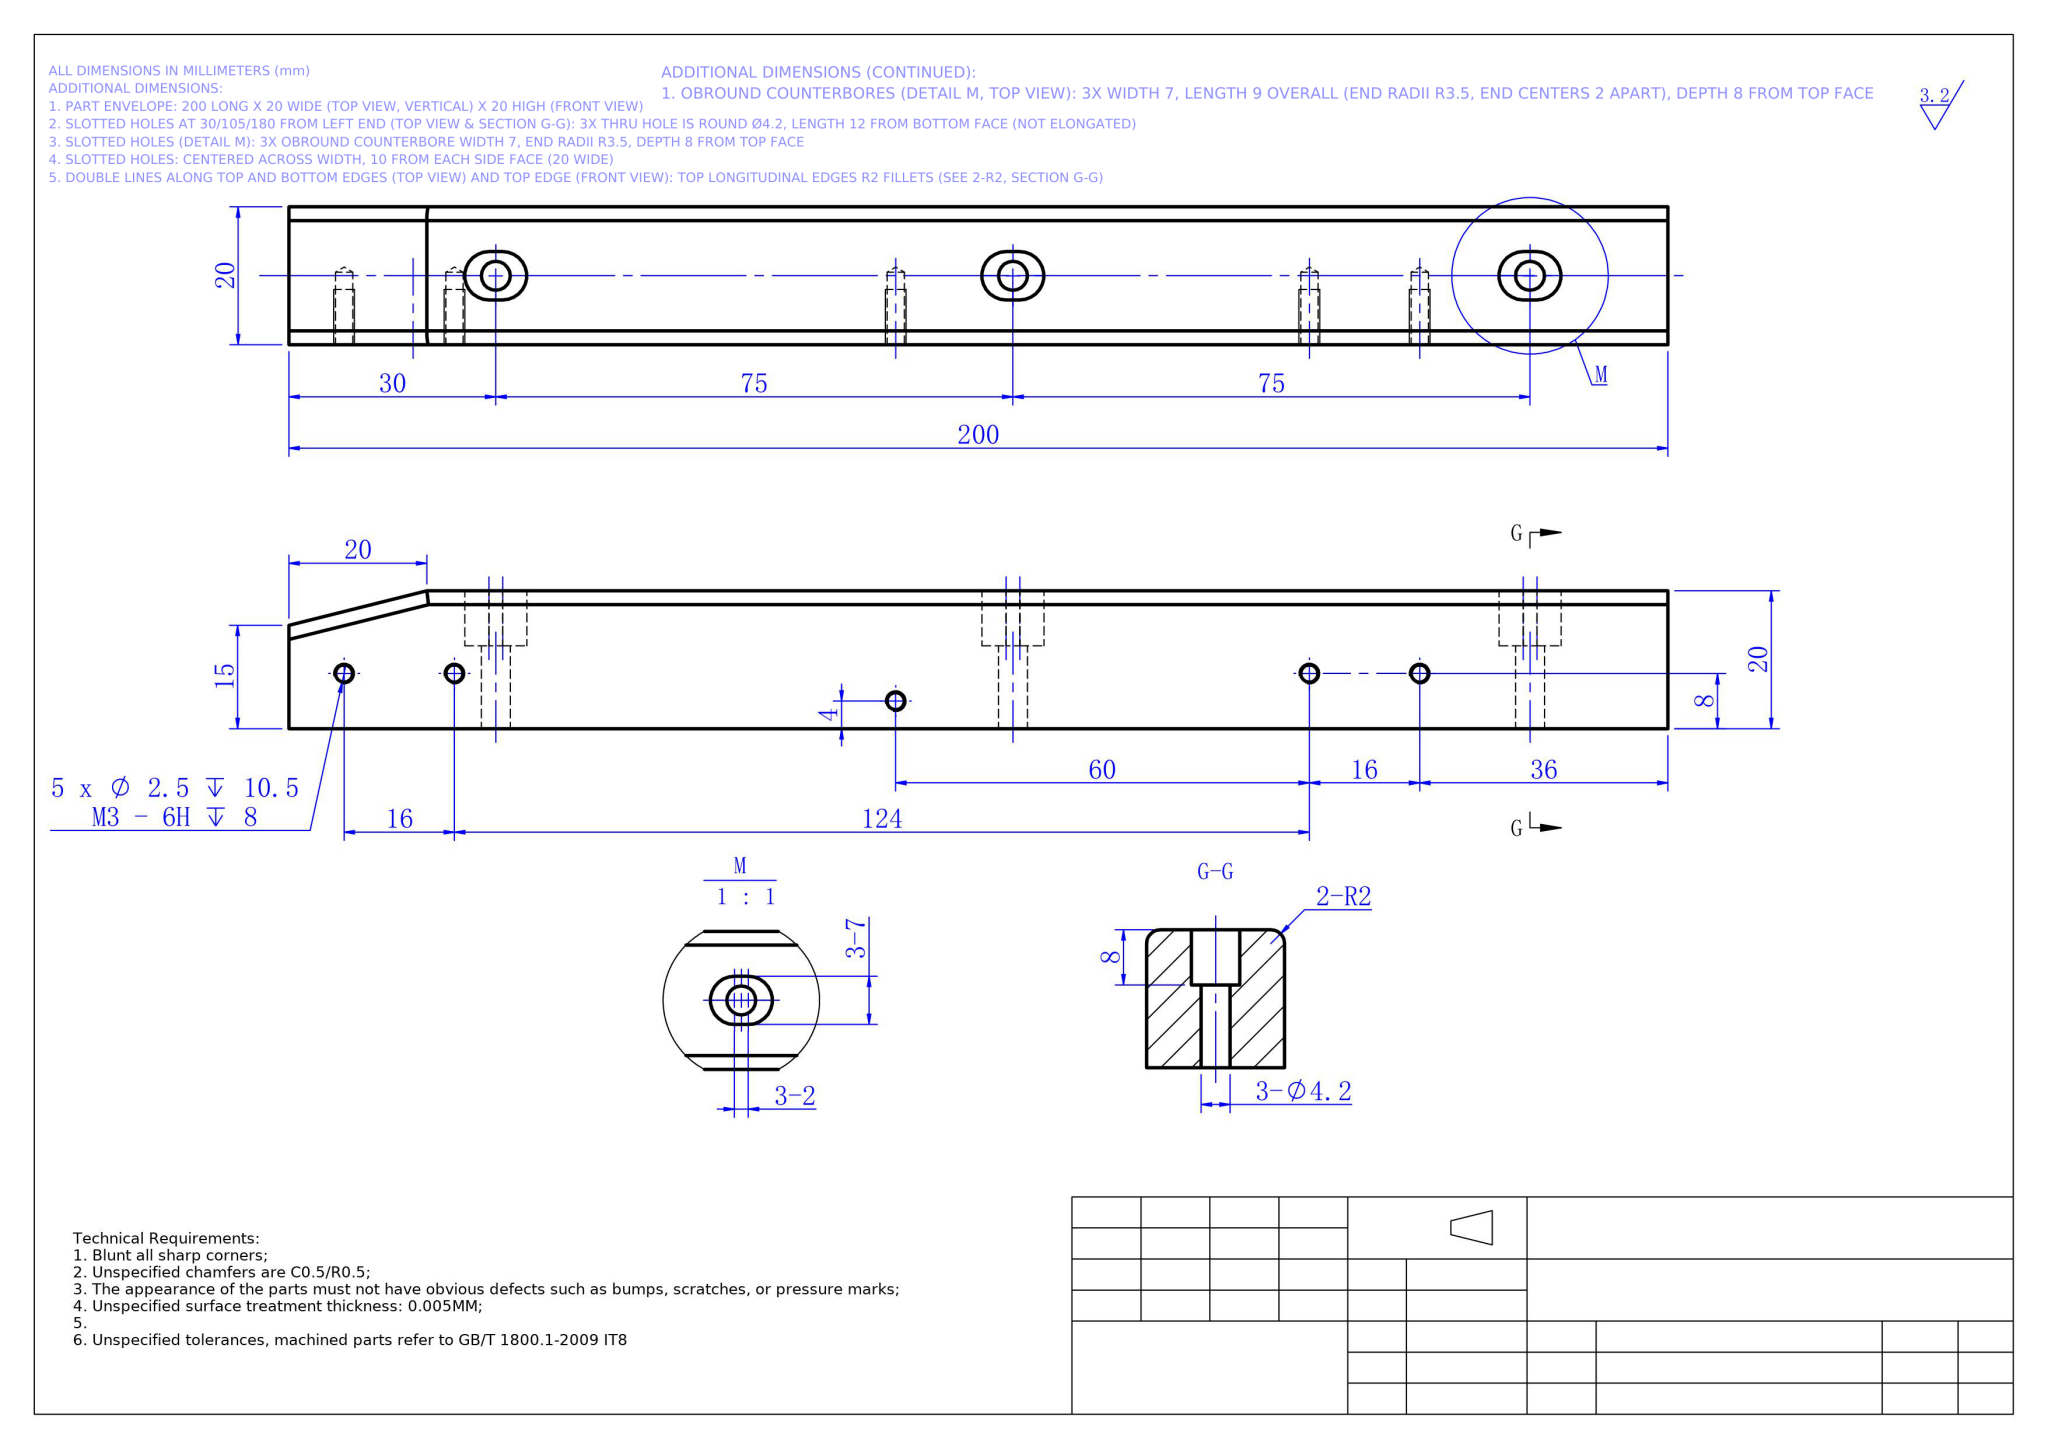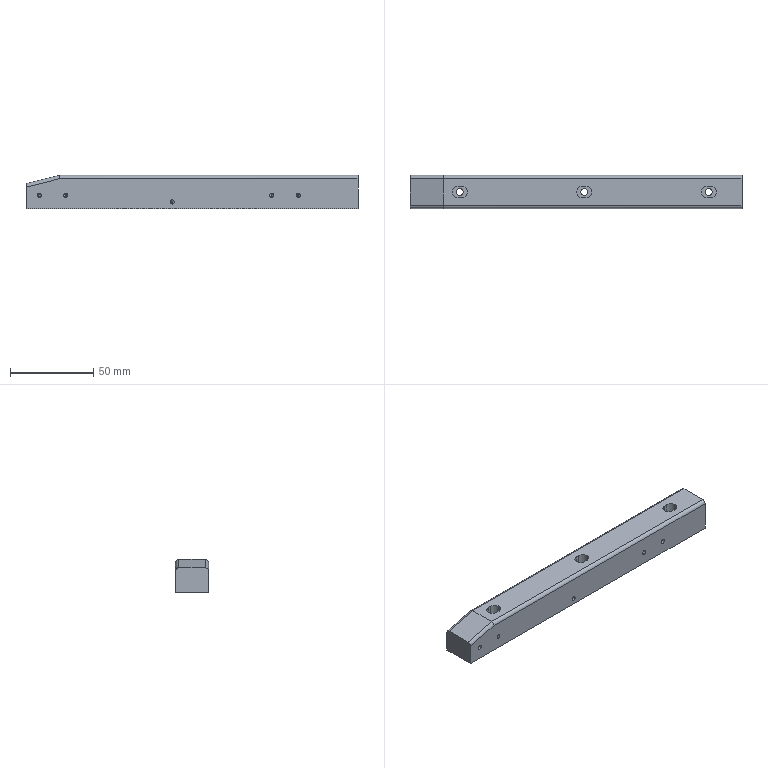Part | NX | mm | 1 solid | 55 faces | box 200 x 20 x 20 mm | volume 76633 mm3 | cylinder 29 | plane 16 | cone 10 | commonest cylinder face diameters 2.5 x10 7 x9 4.2 x6 4 x4